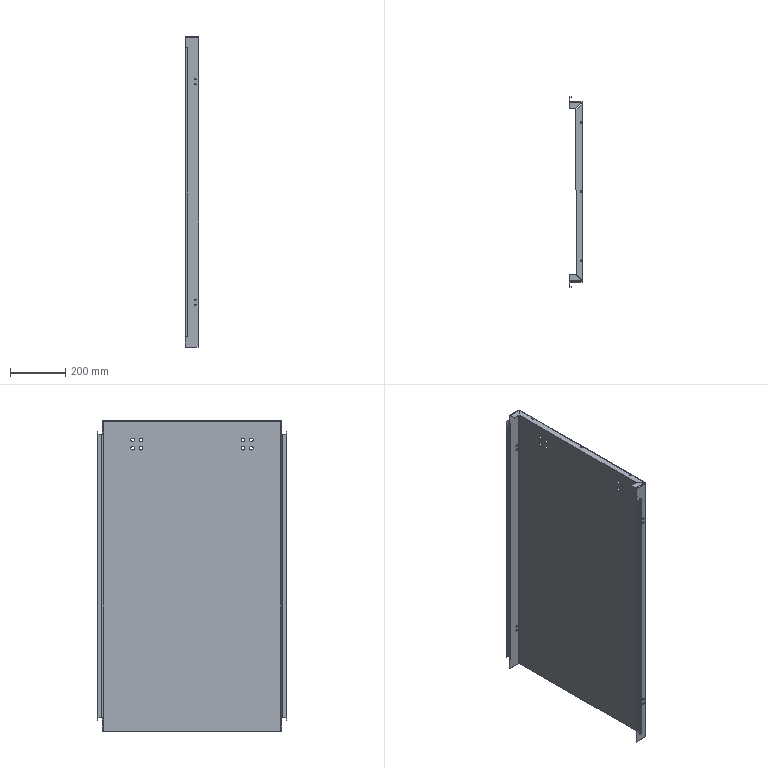Component | SolidWorks | BoxSidePlate01-1 | 1 solid | 148 faces | volume 1356074 mm3 | plane 88 | cylinder 56 | spline 4 | commonest cylinder face diameters 7 x16 13 x16 6 x15 3 x9